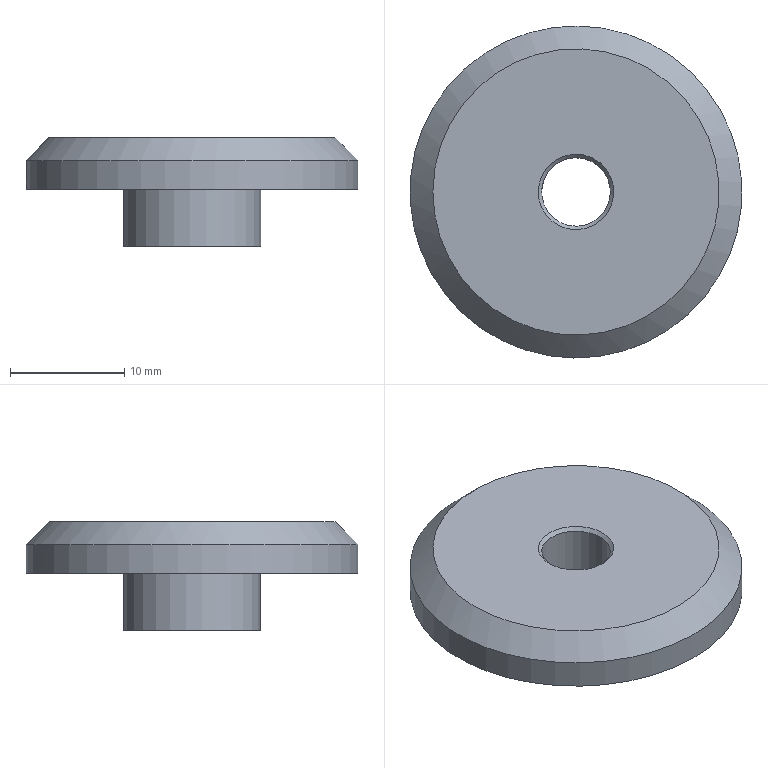Component | NX | CLAMP_BLOCK | 1 solid | 9 faces | box 29 x 29 x 9.5 mm | volume 3094 mm3 | plane 3 | cylinder 3 | cone 3 | commonest cylinder face diameters 29 x1 12 x1 6 x1
STEP:
#1=CARTESIAN_POINT('',(0.,0.,0.));
#2=DIRECTION('',(0.,0.,1.));
#3=DIRECTION('',(1.,0.,0.));
#4=AXIS2_PLACEMENT_3D('',#1,#2,#3);
#5=CARTESIAN_POINT('',(-14.27,0.5229,-167.111));
#6=VERTEX_POINT('',#5);
#7=CARTESIAN_POINT('',(-8.293,0.,-167.111));
#8=DIRECTION('',(0.,0.,-1.));
#9=DIRECTION('',(-0.9962,0.08716,0.));
#10=AXIS2_PLACEMENT_3D('',#7,#8,#9);
#11=CIRCLE('',#10,6.);
#12=CARTESIAN_POINT('',(-8.293,0.,-167.111));
#13=DIRECTION('',(0.,0.,-1.));
#14=DIRECTION('',(-0.9962,0.08716,0.));
#15=AXIS2_PLACEMENT_3D('',#12,#13,#14);
#16=PLANE('',#15);
#17=CARTESIAN_POINT('',(0.,0.));
#18=DIRECTION('',(1.,-0.));
#19=AXIS2_PLACEMENT_2D('',#17,#18);
#20=CIRCLE('',#19,6.);
#21=(GEOMETRIC_REPRESENTATION_CONTEXT(2)PARAMETRIC_REPRESENTATION_CONTEXT()REPRESENTATION_CONTEXT('',''));
#22=DEFINITIONAL_REPRESENTATION('',(#20),#21);
#23=PCURVE('',#16,#22);
#24=CARTESIAN_POINT('',(-8.293,0.,-167.111));
#25=DIRECTION('',(0.,0.,-1.));
#26=DIRECTION('',(-0.9962,0.08716,0.));
#27=AXIS2_PLACEMENT_3D('',#24,#25,#26);
#28=CYLINDRICAL_SURFACE('',#27,6.);
#29=CARTESIAN_POINT('',(0.,0.));
#30=DIRECTION('',(1.,0.));
#31=VECTOR('',#30,1.);
#32=LINE('',#29,#31);
#33=(GEOMETRIC_REPRESENTATION_CONTEXT(2)PARAMETRIC_REPRESENTATION_CONTEXT()REPRESENTATION_CONTEXT('',''));
#34=DEFINITIONAL_REPRESENTATION('',(#32),#33);
#35=PCURVE('',#28,#34);
#36=SURFACE_CURVE('',#11,(#23,#35),.PCURVE_S1.);
#37=EDGE_CURVE('',#6,#6,#36,.T.);
#38=ORIENTED_EDGE('',*,*,#37,.F.);
#39=EDGE_LOOP('',(#38));
#40=FACE_BOUND('',#39,.T.);
#41=CARTESIAN_POINT('',(-22.738,1.264,-167.111));
#42=VERTEX_POINT('',#41);
#43=CARTESIAN_POINT('',(-8.293,0.,-167.111));
#44=DIRECTION('',(0.,0.,1.));
#45=DIRECTION('',(-0.9962,0.08716,0.));
#46=AXIS2_PLACEMENT_3D('',#43,#44,#45);
#47=CIRCLE('',#46,14.5);
#48=CARTESIAN_POINT('',(14.5,-0.));
#49=CARTESIAN_POINT('',(14.5,-25.115));
#50=CARTESIAN_POINT('',(-7.25,-12.557));
#51=CARTESIAN_POINT('',(-29.,-0.));
#52=CARTESIAN_POINT('',(-7.25,12.557));
#53=CARTESIAN_POINT('',(14.5,25.115));
#54=CARTESIAN_POINT('',(14.5,-0.));
#55=(BOUNDED_CURVE()B_SPLINE_CURVE(2,(#48,#49,#50,#51,#52,#53,#54),.UNSPECIFIED.,.T.,.F.)B_SPLINE_CURVE_WITH_KNOTS((1,2,2,2,2,1),(-2.094,0.,2.094,4.189,6.283,8.378),.UNSPECIFIED.)CURVE()GEOMETRIC_REPRESENTATION_ITEM()RATIONAL_B_SPLINE_CURVE((1.,0.5,1.,0.5,1.,0.5,1.))REPRESENTATION_ITEM(''));
#56=(GEOMETRIC_REPRESENTATION_CONTEXT(2)PARAMETRIC_REPRESENTATION_CONTEXT()REPRESENTATION_CONTEXT('',''));
#57=DEFINITIONAL_REPRESENTATION('',(#55),#56);
#58=PCURVE('',#16,#57);
#59=CARTESIAN_POINT('',(-8.293,0.,-162.611));
#60=DIRECTION('',(0.,0.,-1.));
#61=DIRECTION('',(-0.9962,0.08716,0.));
#62=AXIS2_PLACEMENT_3D('',#59,#60,#61);
#63=CYLINDRICAL_SURFACE('',#62,14.5);
#64=CARTESIAN_POINT('',(6.283,4.5));
#65=DIRECTION('',(-1.,0.));
#66=VECTOR('',#65,1.);
#67=LINE('',#64,#66);
#68=(GEOMETRIC_REPRESENTATION_CONTEXT(2)PARAMETRIC_REPRESENTATION_CONTEXT()REPRESENTATION_CONTEXT('',''));
#69=DEFINITIONAL_REPRESENTATION('',(#67),#68);
#70=PCURVE('',#63,#69);
#71=SURFACE_CURVE('',#47,(#58,#70),.PCURVE_S1.);
#72=EDGE_CURVE('',#42,#42,#71,.T.);
#73=ORIENTED_EDGE('',*,*,#72,.F.);
#74=EDGE_LOOP('',(#73));
#75=FACE_BOUND('',#74,.T.);
#76=ADVANCED_FACE('',(#40,#75),#16,.T.);
#77=CARTESIAN_POINT('',(-5.005,-0.2876,-162.611));
#78=VERTEX_POINT('',#77);
#79=CARTESIAN_POINT('',(-8.293,0.,-162.611));
#80=DIRECTION('',(0.,0.,-1.));
#81=DIRECTION('',(0.9962,-0.08716,0.));
#82=AXIS2_PLACEMENT_3D('',#79,#80,#81);
#83=CIRCLE('',#82,3.3);
#84=CARTESIAN_POINT('',(-8.293,0.,-162.611));
#85=DIRECTION('',(0.,0.,1.));
#86=DIRECTION('',(0.9962,-0.08716,0.));
#87=AXIS2_PLACEMENT_3D('',#84,#85,#86);
#88=PLANE('',#87);
#89=CARTESIAN_POINT('',(3.3,0.));
#90=CARTESIAN_POINT('',(3.3,-5.716));
#91=CARTESIAN_POINT('',(-1.65,-2.858));
#92=CARTESIAN_POINT('',(-6.6,0.));
#93=CARTESIAN_POINT('',(-1.65,2.858));
#94=CARTESIAN_POINT('',(3.3,5.716));
#95=CARTESIAN_POINT('',(3.3,0.));
#96=(BOUNDED_CURVE()B_SPLINE_CURVE(2,(#89,#90,#91,#92,#93,#94,#95),.UNSPECIFIED.,.T.,.F.)B_SPLINE_CURVE_WITH_KNOTS((1,2,2,2,2,1),(-2.094,0.,2.094,4.189,6.283,8.378),.UNSPECIFIED.)CURVE()GEOMETRIC_REPRESENTATION_ITEM()RATIONAL_B_SPLINE_CURVE((1.,0.5,1.,0.5,1.,0.5,1.))REPRESENTATION_ITEM(''));
#97=(GEOMETRIC_REPRESENTATION_CONTEXT(2)PARAMETRIC_REPRESENTATION_CONTEXT()REPRESENTATION_CONTEXT('',''));
#98=DEFINITIONAL_REPRESENTATION('',(#96),#97);
#99=PCURVE('',#88,#98);
#100=CARTESIAN_POINT('',(-8.293,0.,-162.911));
#101=DIRECTION('',(0.,0.,1.));
#102=DIRECTION('',(0.9962,-0.08716,0.));
#103=AXIS2_PLACEMENT_3D('',#100,#101,#102);
#104=CONICAL_SURFACE('',#103,3.,0.7854);
#105=CARTESIAN_POINT('',(6.283,0.3));
#106=DIRECTION('',(-1.,0.));
#107=VECTOR('',#106,1.);
#108=LINE('',#105,#107);
#109=(GEOMETRIC_REPRESENTATION_CONTEXT(2)PARAMETRIC_REPRESENTATION_CONTEXT()REPRESENTATION_CONTEXT('',''));
#110=DEFINITIONAL_REPRESENTATION('',(#108),#109);
#111=PCURVE('',#104,#110);
#112=SURFACE_CURVE('',#83,(#99,#111),.PCURVE_S1.);
#113=EDGE_CURVE('',#78,#78,#112,.T.);
#114=ORIENTED_EDGE('',*,*,#113,.T.);
#115=EDGE_LOOP('',(#114));
#116=FACE_BOUND('',#115,.T.);
#117=CARTESIAN_POINT('',(4.16,-1.089,-162.611));
#118=VERTEX_POINT('',#117);
#119=CARTESIAN_POINT('',(-8.293,0.,-162.611));
#120=DIRECTION('',(0.,0.,1.));
#121=DIRECTION('',(0.9962,-0.08716,0.));
#122=AXIS2_PLACEMENT_3D('',#119,#120,#121);
#123=CIRCLE('',#122,12.5);
#124=CARTESIAN_POINT('',(0.,0.));
#125=DIRECTION('',(1.,0.));
#126=AXIS2_PLACEMENT_2D('',#124,#125);
#127=CIRCLE('',#126,12.5);
#128=(GEOMETRIC_REPRESENTATION_CONTEXT(2)PARAMETRIC_REPRESENTATION_CONTEXT()REPRESENTATION_CONTEXT('',''));
#129=DEFINITIONAL_REPRESENTATION('',(#127),#128);
#130=PCURVE('',#88,#129);
#131=CARTESIAN_POINT('',(-8.293,0.,-164.611));
#132=DIRECTION('',(0.,0.,-1.));
#133=DIRECTION('',(-0.9962,0.08716,0.));
#134=AXIS2_PLACEMENT_3D('',#131,#132,#133);
#135=CONICAL_SURFACE('',#134,14.5,0.7854);
#136=CARTESIAN_POINT('',(9.425,-2.));
#137=DIRECTION('',(-1.,0.));
#138=VECTOR('',#137,1.);
#139=LINE('',#136,#138);
#140=(GEOMETRIC_REPRESENTATION_CONTEXT(2)PARAMETRIC_REPRESENTATION_CONTEXT()REPRESENTATION_CONTEXT('',''));
#141=DEFINITIONAL_REPRESENTATION('',(#139),#140);
#142=PCURVE('',#135,#141);
#143=SURFACE_CURVE('',#123,(#130,#142),.PCURVE_S1.);
#144=EDGE_CURVE('',#118,#118,#143,.T.);
#145=ORIENTED_EDGE('',*,*,#144,.T.);
#146=EDGE_LOOP('',(#145));
#147=FACE_BOUND('',#146,.T.);
#148=ADVANCED_FACE('',(#116,#147),#88,.T.);
#149=CARTESIAN_POINT('',(6.152,-1.264,-164.611));
#150=VERTEX_POINT('',#149);
#151=CARTESIAN_POINT('',(-22.738,1.264,-164.611));
#152=VERTEX_POINT('',#151);
#153=CARTESIAN_POINT('',(-8.293,0.,-164.611));
#154=DIRECTION('',(0.,0.,-1.));
#155=DIRECTION('',(0.9962,-0.08716,0.));
#156=AXIS2_PLACEMENT_3D('',#153,#154,#155);
#157=CIRCLE('',#156,14.5);
#158=CARTESIAN_POINT('',(3.142,2.));
#159=DIRECTION('',(1.,0.));
#160=VECTOR('',#159,1.);
#161=LINE('',#158,#160);
#162=(GEOMETRIC_REPRESENTATION_CONTEXT(2)PARAMETRIC_REPRESENTATION_CONTEXT()REPRESENTATION_CONTEXT('',''));
#163=DEFINITIONAL_REPRESENTATION('',(#161),#162);
#164=PCURVE('',#63,#163);
#165=CARTESIAN_POINT('',(3.142,0.));
#166=DIRECTION('',(1.,-0.));
#167=VECTOR('',#166,1.);
#168=LINE('',#165,#167);
#169=(GEOMETRIC_REPRESENTATION_CONTEXT(2)PARAMETRIC_REPRESENTATION_CONTEXT()REPRESENTATION_CONTEXT('',''));
#170=DEFINITIONAL_REPRESENTATION('',(#168),#169);
#171=PCURVE('',#135,#170);
#172=SURFACE_CURVE('',#157,(#164,#171),.PCURVE_S1.);
#173=EDGE_CURVE('',#150,#152,#172,.T.);
#174=ORIENTED_EDGE('',*,*,#173,.T.);
#175=CARTESIAN_POINT('',(-22.738,1.264,-164.611));
#176=CARTESIAN_POINT('',(-22.738,1.264,-167.111));
#177=B_SPLINE_CURVE_WITH_KNOTS('',1,(#175,#176),.UNSPECIFIED.,.F.,.F.,(2,2),(2.,4.5),.PIECEWISE_BEZIER_KNOTS.);
#178=CARTESIAN_POINT('',(6.283,0.));
#179=DIRECTION('',(0.,1.));
#180=VECTOR('',#179,1.);
#181=LINE('',#178,#180);
#182=(GEOMETRIC_REPRESENTATION_CONTEXT(2)PARAMETRIC_REPRESENTATION_CONTEXT()REPRESENTATION_CONTEXT('',''));
#183=DEFINITIONAL_REPRESENTATION('',(#181),#182);
#184=PCURVE('',#63,#183);
#185=CARTESIAN_POINT('',(0.,0.));
#186=DIRECTION('',(0.,1.));
#187=VECTOR('',#186,1.);
#188=LINE('',#185,#187);
#189=(GEOMETRIC_REPRESENTATION_CONTEXT(2)PARAMETRIC_REPRESENTATION_CONTEXT()REPRESENTATION_CONTEXT('',''));
#190=DEFINITIONAL_REPRESENTATION('',(#188),#189);
#191=PCURVE('',#63,#190);
#192=SEAM_CURVE('',#177,(#184,#191),.PCURVE_S1.);
#193=EDGE_CURVE('',#152,#42,#192,.T.);
#194=ORIENTED_EDGE('',*,*,#193,.T.);
#195=ORIENTED_EDGE('',*,*,#72,.T.);
#196=ORIENTED_EDGE('',*,*,#193,.F.);
#197=CARTESIAN_POINT('',(-8.293,0.,-164.611));
#198=DIRECTION('',(0.,0.,-1.));
#199=DIRECTION('',(0.9962,-0.08716,0.));
#200=AXIS2_PLACEMENT_3D('',#197,#198,#199);
#201=CIRCLE('',#200,14.5);
#202=CARTESIAN_POINT('',(-3.142,2.));
#203=DIRECTION('',(1.,0.));
#204=VECTOR('',#203,1.);
#205=LINE('',#202,#204);
#206=(GEOMETRIC_REPRESENTATION_CONTEXT(2)PARAMETRIC_REPRESENTATION_CONTEXT()REPRESENTATION_CONTEXT('',''));
#207=DEFINITIONAL_REPRESENTATION('',(#205),#206);
#208=PCURVE('',#63,#207);
#209=CARTESIAN_POINT('',(3.142,-0.));
#210=DIRECTION('',(1.,0.));
#211=VECTOR('',#210,1.);
#212=LINE('',#209,#211);
#213=(GEOMETRIC_REPRESENTATION_CONTEXT(2)PARAMETRIC_REPRESENTATION_CONTEXT()REPRESENTATION_CONTEXT('',''));
#214=DEFINITIONAL_REPRESENTATION('',(#212),#213);
#215=PCURVE('',#135,#214);
#216=SURFACE_CURVE('',#201,(#208,#215),.PCURVE_S1.);
#217=EDGE_CURVE('',#152,#150,#216,.T.);
#218=ORIENTED_EDGE('',*,*,#217,.T.);
#219=EDGE_LOOP('',(#174,#194,#195,#196,#218));
#220=FACE_BOUND('',#219,.T.);
#221=ADVANCED_FACE('',(#220),#63,.T.);
#222=CARTESIAN_POINT('',(-11.58,0.2876,-172.111));
#223=VERTEX_POINT('',#222);
#224=CARTESIAN_POINT('',(-8.293,0.,-172.111));
#225=DIRECTION('',(0.,0.,1.));
#226=DIRECTION('',(-0.9962,0.08716,0.));
#227=AXIS2_PLACEMENT_3D('',#224,#225,#226);
#228=CIRCLE('',#227,3.3);
#229=CARTESIAN_POINT('',(-8.293,0.,-172.111));
#230=DIRECTION('',(0.,0.,-1.));
#231=DIRECTION('',(-0.9962,0.08716,0.));
#232=AXIS2_PLACEMENT_3D('',#229,#230,#231);
#233=PLANE('',#232);
#234=CARTESIAN_POINT('',(3.3,0.));
#235=CARTESIAN_POINT('',(3.3,-5.716));
#236=CARTESIAN_POINT('',(-1.65,-2.858));
#237=CARTESIAN_POINT('',(-6.6,-0.));
#238=CARTESIAN_POINT('',(-1.65,2.858));
#239=CARTESIAN_POINT('',(3.3,5.716));
#240=CARTESIAN_POINT('',(3.3,0.));
#241=(BOUNDED_CURVE()B_SPLINE_CURVE(2,(#234,#235,#236,#237,#238,#239,#240),.UNSPECIFIED.,.T.,.F.)B_SPLINE_CURVE_WITH_KNOTS((1,2,2,2,2,1),(-2.094,0.,2.094,4.189,6.283,8.378),.UNSPECIFIED.)CURVE()GEOMETRIC_REPRESENTATION_ITEM()RATIONAL_B_SPLINE_CURVE((1.,0.5,1.,0.5,1.,0.5,1.))REPRESENTATION_ITEM(''));
#242=(GEOMETRIC_REPRESENTATION_CONTEXT(2)PARAMETRIC_REPRESENTATION_CONTEXT()REPRESENTATION_CONTEXT('',''));
#243=DEFINITIONAL_REPRESENTATION('',(#241),#242);
#244=PCURVE('',#233,#243);
#245=CARTESIAN_POINT('',(-8.293,0.,-172.111));
#246=DIRECTION('',(0.,0.,-1.));
#247=DIRECTION('',(-0.9962,0.08716,0.));
#248=AXIS2_PLACEMENT_3D('',#245,#246,#247);
#249=CONICAL_SURFACE('',#248,3.3,0.7854);
#250=CARTESIAN_POINT('',(6.283,0.));
#251=DIRECTION('',(-1.,0.));
#252=VECTOR('',#251,1.);
#253=LINE('',#250,#252);
#254=(GEOMETRIC_REPRESENTATION_CONTEXT(2)PARAMETRIC_REPRESENTATION_CONTEXT()REPRESENTATION_CONTEXT('',''));
#255=DEFINITIONAL_REPRESENTATION('',(#253),#254);
#256=PCURVE('',#249,#255);
#257=SURFACE_CURVE('',#228,(#244,#256),.PCURVE_S1.);
#258=EDGE_CURVE('',#223,#223,#257,.T.);
#259=ORIENTED_EDGE('',*,*,#258,.T.);
#260=EDGE_LOOP('',(#259));
#261=FACE_BOUND('',#260,.T.);
#262=CARTESIAN_POINT('',(-14.27,0.5229,-172.111));
#263=VERTEX_POINT('',#262);
#264=CARTESIAN_POINT('',(-8.293,0.,-172.111));
#265=DIRECTION('',(0.,0.,-1.));
#266=DIRECTION('',(-0.9962,0.08716,0.));
#267=AXIS2_PLACEMENT_3D('',#264,#265,#266);
#268=CIRCLE('',#267,6.);
#269=CARTESIAN_POINT('',(0.,0.));
#270=DIRECTION('',(1.,-0.));
#271=AXIS2_PLACEMENT_2D('',#269,#270);
#272=CIRCLE('',#271,6.);
#273=(GEOMETRIC_REPRESENTATION_CONTEXT(2)PARAMETRIC_REPRESENTATION_CONTEXT()REPRESENTATION_CONTEXT('',''));
#274=DEFINITIONAL_REPRESENTATION('',(#272),#273);
#275=PCURVE('',#233,#274);
#276=CARTESIAN_POINT('',(0.,5.));
#277=DIRECTION('',(1.,0.));
#278=VECTOR('',#277,1.);
#279=LINE('',#276,#278);
#280=(GEOMETRIC_REPRESENTATION_CONTEXT(2)PARAMETRIC_REPRESENTATION_CONTEXT()REPRESENTATION_CONTEXT('',''));
#281=DEFINITIONAL_REPRESENTATION('',(#279),#280);
#282=PCURVE('',#28,#281);
#283=SURFACE_CURVE('',#268,(#275,#282),.PCURVE_S1.);
#284=EDGE_CURVE('',#263,#263,#283,.T.);
#285=ORIENTED_EDGE('',*,*,#284,.T.);
#286=EDGE_LOOP('',(#285));
#287=FACE_BOUND('',#286,.T.);
#288=ADVANCED_FACE('',(#261,#287),#233,.T.);
#289=ORIENTED_EDGE('',*,*,#284,.F.);
#290=CARTESIAN_POINT('',(-14.27,0.5229,-167.111));
#291=CARTESIAN_POINT('',(-14.27,0.5229,-172.111));
#292=B_SPLINE_CURVE_WITH_KNOTS('',1,(#290,#291),.UNSPECIFIED.,.F.,.F.,(2,2),(0.,5.),.PIECEWISE_BEZIER_KNOTS.);
#293=CARTESIAN_POINT('',(0.,0.));
#294=DIRECTION('',(0.,1.));
#295=VECTOR('',#294,1.);
#296=LINE('',#293,#295);
#297=(GEOMETRIC_REPRESENTATION_CONTEXT(2)PARAMETRIC_REPRESENTATION_CONTEXT()REPRESENTATION_CONTEXT('',''));
#298=DEFINITIONAL_REPRESENTATION('',(#296),#297);
#299=PCURVE('',#28,#298);
#300=CARTESIAN_POINT('',(6.283,0.));
#301=DIRECTION('',(0.,1.));
#302=VECTOR('',#301,1.);
#303=LINE('',#300,#302);
#304=(GEOMETRIC_REPRESENTATION_CONTEXT(2)PARAMETRIC_REPRESENTATION_CONTEXT()REPRESENTATION_CONTEXT('',''));
#305=DEFINITIONAL_REPRESENTATION('',(#303),#304);
#306=PCURVE('',#28,#305);
#307=SEAM_CURVE('',#292,(#299,#306),.PCURVE_S1.);
#308=EDGE_CURVE('',#6,#263,#307,.T.);
#309=ORIENTED_EDGE('',*,*,#308,.F.);
#310=ORIENTED_EDGE('',*,*,#37,.T.);
#311=ORIENTED_EDGE('',*,*,#308,.T.);
#312=EDGE_LOOP('',(#289,#309,#310,#311));
#313=FACE_BOUND('',#312,.T.);
#314=ADVANCED_FACE('',(#313),#28,.T.);
#315=ORIENTED_EDGE('',*,*,#144,.F.);
#316=CARTESIAN_POINT('',(4.16,-1.089,-162.611));
#317=CARTESIAN_POINT('',(6.152,-1.264,-164.611));
#318=B_SPLINE_CURVE_WITH_KNOTS('',1,(#316,#317),.UNSPECIFIED.,.F.,.F.,(2,2),(-2.828,0.),.PIECEWISE_BEZIER_KNOTS.);
#319=CARTESIAN_POINT('',(9.425,0.));
#320=DIRECTION('',(0.,1.));
#321=VECTOR('',#320,1.);
#322=LINE('',#319,#321);
#323=(GEOMETRIC_REPRESENTATION_CONTEXT(2)PARAMETRIC_REPRESENTATION_CONTEXT()REPRESENTATION_CONTEXT('',''));
#324=DEFINITIONAL_REPRESENTATION('',(#322),#323);
#325=PCURVE('',#135,#324);
#326=CARTESIAN_POINT('',(3.142,0.));
#327=DIRECTION('',(0.,1.));
#328=VECTOR('',#327,1.);
#329=LINE('',#326,#328);
#330=(GEOMETRIC_REPRESENTATION_CONTEXT(2)PARAMETRIC_REPRESENTATION_CONTEXT()REPRESENTATION_CONTEXT('',''));
#331=DEFINITIONAL_REPRESENTATION('',(#329),#330);
#332=PCURVE('',#135,#331);
#333=SEAM_CURVE('',#318,(#325,#332),.PCURVE_S1.);
#334=EDGE_CURVE('',#118,#150,#333,.T.);
#335=ORIENTED_EDGE('',*,*,#334,.T.);
#336=ORIENTED_EDGE('',*,*,#217,.F.);
#337=ORIENTED_EDGE('',*,*,#173,.F.);
#338=ORIENTED_EDGE('',*,*,#334,.F.);
#339=EDGE_LOOP('',(#315,#335,#336,#337,#338));
#340=FACE_BOUND('',#339,.T.);
#341=ADVANCED_FACE('',(#340),#135,.T.);
#342=CARTESIAN_POINT('',(-5.304,-0.2615,-162.911));
#343=VERTEX_POINT('',#342);
#344=CARTESIAN_POINT('',(-8.293,0.,-162.911));
#345=DIRECTION('',(0.,0.,1.));
#346=DIRECTION('',(0.9962,-0.08716,0.));
#347=AXIS2_PLACEMENT_3D('',#344,#345,#346);
#348=CIRCLE('',#347,3.);
#349=CARTESIAN_POINT('',(-8.293,0.,-172.111));
#350=DIRECTION('',(0.,0.,1.));
#351=DIRECTION('',(0.9962,-0.08716,0.));
#352=AXIS2_PLACEMENT_3D('',#349,#350,#351);
#353=CYLINDRICAL_SURFACE('',#352,3.);
#354=CARTESIAN_POINT('',(0.,9.2));
#355=DIRECTION('',(1.,0.));
#356=VECTOR('',#355,1.);
#357=LINE('',#354,#356);
#358=(GEOMETRIC_REPRESENTATION_CONTEXT(2)PARAMETRIC_REPRESENTATION_CONTEXT()REPRESENTATION_CONTEXT('',''));
#359=DEFINITIONAL_REPRESENTATION('',(#357),#358);
#360=PCURVE('',#353,#359);
#361=CARTESIAN_POINT('',(0.,0.));
#362=DIRECTION('',(1.,0.));
#363=VECTOR('',#362,1.);
#364=LINE('',#361,#363);
#365=(GEOMETRIC_REPRESENTATION_CONTEXT(2)PARAMETRIC_REPRESENTATION_CONTEXT()REPRESENTATION_CONTEXT('',''));
#366=DEFINITIONAL_REPRESENTATION('',(#364),#365);
#367=PCURVE('',#104,#366);
#368=SURFACE_CURVE('',#348,(#360,#367),.PCURVE_S1.);
#369=EDGE_CURVE('',#343,#343,#368,.T.);
#370=ORIENTED_EDGE('',*,*,#369,.F.);
#371=CARTESIAN_POINT('',(-5.304,-0.2615,-171.811));
#372=VERTEX_POINT('',#371);
#373=CARTESIAN_POINT('',(-5.304,-0.2615,-171.811));
#374=CARTESIAN_POINT('',(-5.304,-0.2615,-162.911));
#375=B_SPLINE_CURVE_WITH_KNOTS('',1,(#373,#374),.UNSPECIFIED.,.F.,.F.,(2,2),(0.3,9.2),.PIECEWISE_BEZIER_KNOTS.);
#376=CARTESIAN_POINT('',(0.,0.));
#377=DIRECTION('',(0.,1.));
#378=VECTOR('',#377,1.);
#379=LINE('',#376,#378);
#380=(GEOMETRIC_REPRESENTATION_CONTEXT(2)PARAMETRIC_REPRESENTATION_CONTEXT()REPRESENTATION_CONTEXT('',''));
#381=DEFINITIONAL_REPRESENTATION('',(#379),#380);
#382=PCURVE('',#353,#381);
#383=CARTESIAN_POINT('',(6.283,0.));
#384=DIRECTION('',(0.,1.));
#385=VECTOR('',#384,1.);
#386=LINE('',#383,#385);
#387=(GEOMETRIC_REPRESENTATION_CONTEXT(2)PARAMETRIC_REPRESENTATION_CONTEXT()REPRESENTATION_CONTEXT('',''));
#388=DEFINITIONAL_REPRESENTATION('',(#386),#387);
#389=PCURVE('',#353,#388);
#390=SEAM_CURVE('',#375,(#382,#389),.PCURVE_S1.);
#391=EDGE_CURVE('',#372,#343,#390,.T.);
#392=ORIENTED_EDGE('',*,*,#391,.F.);
#393=CARTESIAN_POINT('',(-11.281,0.2615,-171.811));
#394=VERTEX_POINT('',#393);
#395=CARTESIAN_POINT('',(-8.293,0.,-171.811));
#396=DIRECTION('',(0.,0.,-1.));
#397=DIRECTION('',(-0.9962,0.08716,0.));
#398=AXIS2_PLACEMENT_3D('',#395,#396,#397);
#399=CIRCLE('',#398,3.);
#400=CARTESIAN_POINT('',(3.142,0.3));
#401=DIRECTION('',(-1.,0.));
#402=VECTOR('',#401,1.);
#403=LINE('',#400,#402);
#404=(GEOMETRIC_REPRESENTATION_CONTEXT(2)PARAMETRIC_REPRESENTATION_CONTEXT()REPRESENTATION_CONTEXT('',''));
#405=DEFINITIONAL_REPRESENTATION('',(#403),#404);
#406=PCURVE('',#353,#405);
#407=CARTESIAN_POINT('',(0.,-0.3));
#408=DIRECTION('',(1.,0.));
#409=VECTOR('',#408,1.);
#410=LINE('',#407,#409);
#411=(GEOMETRIC_REPRESENTATION_CONTEXT(2)PARAMETRIC_REPRESENTATION_CONTEXT()REPRESENTATION_CONTEXT('',''));
#412=DEFINITIONAL_REPRESENTATION('',(#410),#411);
#413=PCURVE('',#249,#412);
#414=SURFACE_CURVE('',#399,(#406,#413),.PCURVE_S1.);
#415=EDGE_CURVE('',#394,#372,#414,.T.);
#416=ORIENTED_EDGE('',*,*,#415,.F.);
#417=CARTESIAN_POINT('',(-8.293,0.,-171.811));
#418=DIRECTION('',(0.,0.,-1.));
#419=DIRECTION('',(-0.9962,0.08716,0.));
#420=AXIS2_PLACEMENT_3D('',#417,#418,#419);
#421=CIRCLE('',#420,3.);
#422=CARTESIAN_POINT('',(9.425,0.3));
#423=DIRECTION('',(-1.,0.));
#424=VECTOR('',#423,1.);
#425=LINE('',#422,#424);
#426=(GEOMETRIC_REPRESENTATION_CONTEXT(2)PARAMETRIC_REPRESENTATION_CONTEXT()REPRESENTATION_CONTEXT('',''));
#427=DEFINITIONAL_REPRESENTATION('',(#425),#426);
#428=PCURVE('',#353,#427);
#429=CARTESIAN_POINT('',(0.,-0.3));
#430=DIRECTION('',(1.,0.));
#431=VECTOR('',#430,1.);
#432=LINE('',#429,#431);
#433=(GEOMETRIC_REPRESENTATION_CONTEXT(2)PARAMETRIC_REPRESENTATION_CONTEXT()REPRESENTATION_CONTEXT('',''));
#434=DEFINITIONAL_REPRESENTATION('',(#432),#433);
#435=PCURVE('',#249,#434);
#436=SURFACE_CURVE('',#421,(#428,#435),.PCURVE_S1.);
#437=EDGE_CURVE('',#372,#394,#436,.T.);
#438=ORIENTED_EDGE('',*,*,#437,.F.);
#439=ORIENTED_EDGE('',*,*,#391,.T.);
#440=EDGE_LOOP('',(#370,#392,#416,#438,#439));
#441=FACE_BOUND('',#440,.F.);
#442=ADVANCED_FACE('',(#441),#353,.F.);
#443=ORIENTED_EDGE('',*,*,#437,.T.);
#444=CARTESIAN_POINT('',(-11.281,0.2615,-171.811));
#445=CARTESIAN_POINT('',(-11.58,0.2876,-172.111));
#446=B_SPLINE_CURVE_WITH_KNOTS('',1,(#444,#445),.UNSPECIFIED.,.F.,.F.,(2,2),(-0.4243,0.),.PIECEWISE_BEZIER_KNOTS.);
#447=CARTESIAN_POINT('',(6.283,0.));
#448=DIRECTION('',(0.,1.));
#449=VECTOR('',#448,1.);
#450=LINE('',#447,#449);
#451=(GEOMETRIC_REPRESENTATION_CONTEXT(2)PARAMETRIC_REPRESENTATION_CONTEXT()REPRESENTATION_CONTEXT('',''));
#452=DEFINITIONAL_REPRESENTATION('',(#450),#451);
#453=PCURVE('',#249,#452);
#454=CARTESIAN_POINT('',(0.,0.));
#455=DIRECTION('',(0.,1.));
#456=VECTOR('',#455,1.);
#457=LINE('',#454,#456);
#458=(GEOMETRIC_REPRESENTATION_CONTEXT(2)PARAMETRIC_REPRESENTATION_CONTEXT()REPRESENTATION_CONTEXT('',''));
#459=DEFINITIONAL_REPRESENTATION('',(#457),#458);
#460=PCURVE('',#249,#459);
#461=SEAM_CURVE('',#446,(#453,#460),.PCURVE_S1.);
#462=EDGE_CURVE('',#394,#223,#461,.T.);
#463=ORIENTED_EDGE('',*,*,#462,.T.);
#464=ORIENTED_EDGE('',*,*,#258,.T.);
#465=ORIENTED_EDGE('',*,*,#462,.F.);
#466=ORIENTED_EDGE('',*,*,#415,.T.);
#467=EDGE_LOOP('',(#443,#463,#464,#465,#466));
#468=FACE_BOUND('',#467,.F.);
#469=ADVANCED_FACE('',(#468),#249,.F.);
#470=ORIENTED_EDGE('',*,*,#113,.T.);
#471=CARTESIAN_POINT('',(-5.304,-0.2615,-162.911));
#472=CARTESIAN_POINT('',(-5.005,-0.2876,-162.611));
#473=B_SPLINE_CURVE_WITH_KNOTS('',1,(#471,#472),.UNSPECIFIED.,.F.,.F.,(2,2),(0.,0.4243),.PIECEWISE_BEZIER_KNOTS.);
#474=CARTESIAN_POINT('',(0.,0.));
#475=DIRECTION('',(0.,1.));
#476=VECTOR('',#475,1.);
#477=LINE('',#474,#476);
#478=(GEOMETRIC_REPRESENTATION_CONTEXT(2)PARAMETRIC_REPRESENTATION_CONTEXT()REPRESENTATION_CONTEXT('',''));
#479=DEFINITIONAL_REPRESENTATION('',(#477),#478);
#480=PCURVE('',#104,#479);
#481=CARTESIAN_POINT('',(6.283,0.));
#482=DIRECTION('',(0.,1.));
#483=VECTOR('',#482,1.);
#484=LINE('',#481,#483);
#485=(GEOMETRIC_REPRESENTATION_CONTEXT(2)PARAMETRIC_REPRESENTATION_CONTEXT()REPRESENTATION_CONTEXT('',''));
#486=DEFINITIONAL_REPRESENTATION('',(#484),#485);
#487=PCURVE('',#104,#486);
#488=SEAM_CURVE('',#473,(#480,#487),.PCURVE_S1.);
#489=EDGE_CURVE('',#343,#78,#488,.T.);
#490=ORIENTED_EDGE('',*,*,#489,.F.);
#491=ORIENTED_EDGE('',*,*,#369,.T.);
#492=ORIENTED_EDGE('',*,*,#489,.T.);
#493=EDGE_LOOP('',(#470,#490,#491,#492));
#494=FACE_BOUND('',#493,.F.);
#495=ADVANCED_FACE('',(#494),#104,.F.);
#496=CLOSED_SHELL('',(#76,#148,#221,#288,#314,#341,#442,#469,#495));
#497=MANIFOLD_SOLID_BREP('',#496);
#498=(LENGTH_UNIT()NAMED_UNIT(*)SI_UNIT(.MILLI.,.METRE.));
#499=UNCERTAINTY_MEASURE_WITH_UNIT(LENGTH_MEASURE(0.00001),#498,'','');
#500=(NAMED_UNIT(*)PLANE_ANGLE_UNIT()SI_UNIT($,.RADIAN.));
#501=(NAMED_UNIT(*)SI_UNIT($,.STERADIAN.)SOLID_ANGLE_UNIT());
#502=(GEOMETRIC_REPRESENTATION_CONTEXT(3)GLOBAL_UNCERTAINTY_ASSIGNED_CONTEXT((#499))GLOBAL_UNIT_ASSIGNED_CONTEXT((#498,#500,#501))REPRESENTATION_CONTEXT('',''));
#503=ADVANCED_BREP_SHAPE_REPRESENTATION('',(#4,#497),#502);